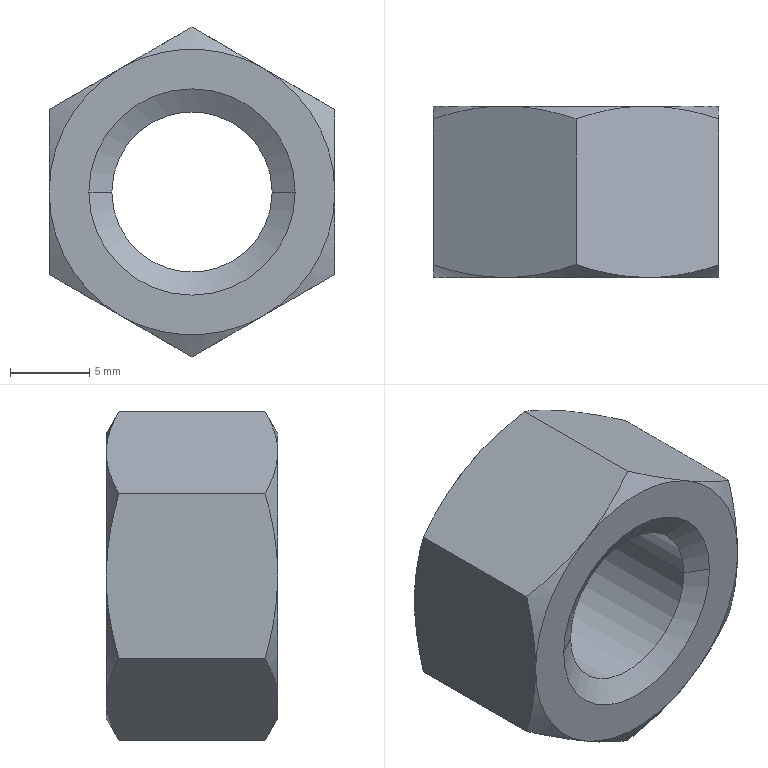Component | SolidWorks | GB_T6170-2015[Type1HexNutM12]-1 | 1 solid | 26 faces | box 18 x 10.8 x 20.78 mm | volume 2109 mm3 | cone 16 | plane 8 | cylinder 2 | commonest cylinder face diameters 10.106 x2
build123d program:
from build123d import *

# Parameters (mm, degrees)
SKETCH3_R           = 5.053
BOSS_EXTRUDE1_DEPTH = 10.8
SKETCH5_R           = 15.023
SKETCH5_R_2         = 9
CUT_EXTRUDE1_DEPTH  = 2.16
CUT_EXTRUDE1_DRAFT  = -60
SKETCH7_R           = 15.023
SKETCH7_R_2         = 9
CUT_EXTRUDE2_DEPTH  = 2.16
CUT_EXTRUDE2_DRAFT  = -60


with BuildPart() as part:
    # Sketch3 → Boss-Extrude1 (new body)
    with BuildSketch(Plane.XY):
        Polygon((0, 10.392), (-9, 5.196), (-9, -5.196), (0, -10.392), (9, -5.196), (9, 5.196), align=None)
        Circle(SKETCH3_R, mode=Mode.SUBTRACT)
    extrude(amount=-BOSS_EXTRUDE1_DEPTH)

    # Sketch4 → Cut-Revolve1 (revolve, cut)
    with BuildSketch(Plane(origin=(0, 0, 0), x_dir=(0, 0, -1), z_dir=(1, 0, 0)), mode=Mode.PRIVATE) as cut_revolve1_sk:
        Polygon((0, 6.5), (0.8355, 5.053), (0.8355, 0), (0, 0), align=None)
        Polygon((10.8, 0), (10.8, 6.5), (9.964, 5.053), (9.964, 0), align=None)
    revolve(cut_revolve1_sk.sketch.rotate(Axis((0, 0, 0), (0, 0, -1)), 90), axis=Axis((0, 0, 0), (0, 0, -1)), mode=Mode.SUBTRACT)


with BuildPart() as cut_extrude1_tool:
    # Sketch5 → Cut-Extrude1 (with draft: the straight prism first)
    with BuildSketch(Plane.XY):
        Circle(SKETCH5_R)
        Circle(SKETCH5_R_2, mode=Mode.SUBTRACT)
    extrude(amount=-CUT_EXTRUDE1_DEPTH)
    # Cut-Extrude1: the draft: its side faces are tilted about the plane it starts from
    cut_extrude1_sides = [cut_extrude1_tool.faces().sort_by_distance(p)[0] for p in [
        (-15.023, 0, -1.08),
        (-9, 0, -1.08),
    ]]
    draft(cut_extrude1_sides, Plane.XY, CUT_EXTRUDE1_DRAFT)


with BuildPart() as part_1:
    add(part.part)

    # Cut-Extrude1: cut by cut_extrude1_tool
    add(cut_extrude1_tool.part, mode=Mode.SUBTRACT)


with BuildPart() as cut_extrude2_tool:
    # Sketch7 → Cut-Extrude2 (with draft: the straight prism first)
    with BuildSketch(Plane(origin=(0, 0, -10.8), x_dir=(-1, 0, 0), z_dir=(0, 0, -1))):
        Circle(SKETCH7_R)
        Circle(SKETCH7_R_2, mode=Mode.SUBTRACT)
    extrude(amount=-CUT_EXTRUDE2_DEPTH)
    # Cut-Extrude2: the draft: its side faces are tilted about the plane it starts from
    cut_extrude2_sides = [cut_extrude2_tool.faces().sort_by_distance(p)[0] for p in [
        (15.023, 0, -9.72),
        (9, 0, -9.72),
    ]]
    draft(cut_extrude2_sides, Plane(origin=(0, 0, -10.8), x_dir=(-1, 0, 0), z_dir=(0, 0, -1)), CUT_EXTRUDE2_DRAFT)


with BuildPart() as part_2:
    add(part_1.part)

    # Cut-Extrude2: cut by cut_extrude2_tool
    add(cut_extrude2_tool.part, mode=Mode.SUBTRACT)


solid = part_2.part

# Placed as in the assembly
solid = solid.moved(Location((128, 179.606, 0), (90, 0, 0)))
STEP:
#1=COLOUR_RGB('',0.7922,0.8196,0.9333);
#2=FILL_AREA_STYLE_COLOUR('',#1);
#3=FILL_AREA_STYLE('',(#2));
#4=SURFACE_STYLE_FILL_AREA(#3);
#5=SURFACE_SIDE_STYLE('',(#4));
#6=SURFACE_STYLE_USAGE(.BOTH.,#5);
#7=PRESENTATION_STYLE_ASSIGNMENT((#6));
#8=CARTESIAN_POINT('',(4.84,7.463,0.));
#9=VERTEX_POINT('',#8);
#10=CARTESIAN_POINT('',(5.238,7.463,0.));
#11=VERTEX_POINT('',#10);
#12=CARTESIAN_POINT('',(5.039,7.463,0.));
#13=DIRECTION('',(0.,-1.,0.));
#14=DIRECTION('',(1.,0.,0.));
#15=AXIS2_PLACEMENT_3D('',#12,#13,#14);
#16=CIRCLE('',#15,0.1989);
#17=EDGE_CURVE('',#9,#11,#16,.T.);
#18=ORIENTED_EDGE('',*,*,#17,.T.);
#19=CARTESIAN_POINT('',(5.295,7.496,0.));
#20=VERTEX_POINT('',#19);
#21=CARTESIAN_POINT('',(5.295,7.496,0.));
#22=DIRECTION('',(0.866,0.5,0.));
#23=VECTOR('',#22,39.37);
#24=LINE('',#21,#23);
#25=EDGE_CURVE('',#11,#20,#24,.T.);
#26=ORIENTED_EDGE('',*,*,#25,.T.);
#27=CARTESIAN_POINT('',(4.783,7.496,0.));
#28=VERTEX_POINT('',#27);
#29=CARTESIAN_POINT('',(5.039,7.496,0.));
#30=DIRECTION('',(0.,-1.,0.));
#31=DIRECTION('',(1.,0.,0.));
#32=AXIS2_PLACEMENT_3D('',#29,#30,#31);
#33=CIRCLE('',#32,0.2559);
#34=EDGE_CURVE('',#28,#20,#33,.T.);
#35=ORIENTED_EDGE('',*,*,#34,.F.);
#36=CARTESIAN_POINT('',(4.783,7.496,0.));
#37=DIRECTION('',(-0.866,0.5,0.));
#38=VECTOR('',#37,39.37);
#39=LINE('',#36,#38);
#40=EDGE_CURVE('',#9,#28,#39,.T.);
#41=ORIENTED_EDGE('',*,*,#40,.F.);
#42=EDGE_LOOP('',(#18,#26,#35,#41));
#43=FACE_OUTER_BOUND('',#42,.T.);
#44=CARTESIAN_POINT('',(5.039,7.496,0.));
#45=DIRECTION('',(0.,1.,0.));
#46=DIRECTION('',(-1.,0.,0.));
#47=AXIS2_PLACEMENT_3D('',#44,#45,#46);
#48=CONICAL_SURFACE('',#47,0.2559,1.047);
#49=ADVANCED_FACE('',(#43),#48,.F.);
#50=CARTESIAN_POINT('',(4.84,7.104,0.));
#51=VERTEX_POINT('',#50);
#52=CARTESIAN_POINT('',(5.238,7.104,0.));
#53=VERTEX_POINT('',#52);
#54=CARTESIAN_POINT('',(5.039,7.104,0.));
#55=DIRECTION('',(0.,-1.,0.));
#56=DIRECTION('',(1.,0.,0.));
#57=AXIS2_PLACEMENT_3D('',#54,#55,#56);
#58=CIRCLE('',#57,0.1989);
#59=EDGE_CURVE('',#51,#53,#58,.T.);
#60=ORIENTED_EDGE('',*,*,#59,.F.);
#61=CARTESIAN_POINT('',(4.783,7.071,0.));
#62=VERTEX_POINT('',#61);
#63=CARTESIAN_POINT('',(4.84,7.104,0.));
#64=DIRECTION('',(-0.866,-0.5,0.));
#65=VECTOR('',#64,39.37);
#66=LINE('',#63,#65);
#67=EDGE_CURVE('',#51,#62,#66,.T.);
#68=ORIENTED_EDGE('',*,*,#67,.T.);
#69=CARTESIAN_POINT('',(5.295,7.071,0.));
#70=VERTEX_POINT('',#69);
#71=CARTESIAN_POINT('',(5.039,7.071,0.));
#72=DIRECTION('',(0.,-1.,0.));
#73=DIRECTION('',(1.,0.,0.));
#74=AXIS2_PLACEMENT_3D('',#71,#72,#73);
#75=CIRCLE('',#74,0.2559);
#76=EDGE_CURVE('',#62,#70,#75,.T.);
#77=ORIENTED_EDGE('',*,*,#76,.T.);
#78=CARTESIAN_POINT('',(5.238,7.104,0.));
#79=DIRECTION('',(0.866,-0.5,0.));
#80=VECTOR('',#79,39.37);
#81=LINE('',#78,#80);
#82=EDGE_CURVE('',#53,#70,#81,.T.);
#83=ORIENTED_EDGE('',*,*,#82,.F.);
#84=EDGE_LOOP('',(#60,#68,#77,#83));
#85=FACE_OUTER_BOUND('',#84,.T.);
#86=CARTESIAN_POINT('',(5.039,7.104,0.));
#87=DIRECTION('',(0.,-1.,0.));
#88=DIRECTION('',(1.,0.,0.));
#89=AXIS2_PLACEMENT_3D('',#86,#87,#88);
#90=CONICAL_SURFACE('',#89,0.1989,1.047);
#91=ADVANCED_FACE('',(#85),#90,.F.);
#92=ORIENTED_EDGE('',*,*,#17,.F.);
#93=CARTESIAN_POINT('',(4.84,7.496,0.));
#94=DIRECTION('',(0.,-1.,0.));
#95=VECTOR('',#94,39.37);
#96=LINE('',#93,#95);
#97=EDGE_CURVE('',#9,#51,#96,.T.);
#98=ORIENTED_EDGE('',*,*,#97,.T.);
#99=ORIENTED_EDGE('',*,*,#59,.T.);
#100=CARTESIAN_POINT('',(5.238,7.496,0.));
#101=DIRECTION('',(0.,-1.,0.));
#102=VECTOR('',#101,39.37);
#103=LINE('',#100,#102);
#104=EDGE_CURVE('',#11,#53,#103,.T.);
#105=ORIENTED_EDGE('',*,*,#104,.F.);
#106=EDGE_LOOP('',(#92,#98,#99,#105));
#107=FACE_OUTER_BOUND('',#106,.T.);
#108=CARTESIAN_POINT('',(5.039,7.496,0.));
#109=DIRECTION('',(0.,-1.,0.));
#110=DIRECTION('',(1.,0.,0.));
#111=AXIS2_PLACEMENT_3D('',#108,#109,#110);
#112=CYLINDRICAL_SURFACE('',#111,0.1989);
#113=ADVANCED_FACE('',(#107),#112,.F.);
#114=CARTESIAN_POINT('',(5.394,7.465,0.2046));
#115=VERTEX_POINT('',#114);
#116=CARTESIAN_POINT('',(5.394,7.103,0.2046));
#117=VERTEX_POINT('',#116);
#118=CARTESIAN_POINT('',(5.394,7.496,0.2046));
#119=DIRECTION('',(0.,-1.,0.));
#120=VECTOR('',#119,39.37);
#121=LINE('',#118,#120);
#122=EDGE_CURVE('',#115,#117,#121,.T.);
#123=ORIENTED_EDGE('',*,*,#122,.F.);
#124=CARTESIAN_POINT('',(5.217,7.496,0.3069));
#125=VERTEX_POINT('',#124);
#126=CARTESIAN_POINT('',(5.394,7.465,0.2046));
#127=CARTESIAN_POINT('',(5.365,7.474,0.2213));
#128=CARTESIAN_POINT('',(5.336,7.482,0.2382));
#129=CARTESIAN_POINT('',(5.277,7.493,0.2722));
#130=CARTESIAN_POINT('',(5.247,7.496,0.2894));
#131=CARTESIAN_POINT('',(5.217,7.496,0.3069));
#132=B_SPLINE_CURVE_WITH_KNOTS('',3,(#126,#127,#128,#129,#130,#131),.UNSPECIFIED.,.F.,.F.,(4,2,4),(0.00000024,0.002629,0.005258),.UNSPECIFIED.);
#133=EDGE_CURVE('',#115,#125,#132,.T.);
#134=ORIENTED_EDGE('',*,*,#133,.T.);
#135=CARTESIAN_POINT('',(5.039,7.465,0.4091));
#136=VERTEX_POINT('',#135);
#137=CARTESIAN_POINT('',(5.217,7.496,0.3069));
#138=CARTESIAN_POINT('',(5.201,7.496,0.3155));
#139=CARTESIAN_POINT('',(5.186,7.496,0.3243));
#140=CARTESIAN_POINT('',(5.157,7.493,0.3415));
#141=CARTESIAN_POINT('',(5.142,7.49,0.3501));
#142=CARTESIAN_POINT('',(5.097,7.482,0.3756));
#143=CARTESIAN_POINT('',(5.068,7.474,0.3925));
#144=CARTESIAN_POINT('',(5.039,7.465,0.4091));
#145=B_SPLINE_CURVE_WITH_KNOTS('',3,(#137,#138,#139,#140,#141,#142,#143,#144),.UNSPECIFIED.,.F.,.F.,(4,2,2,4),(0.005258,0.006567,0.007877,0.0105),.UNSPECIFIED.);
#146=EDGE_CURVE('',#125,#136,#145,.T.);
#147=ORIENTED_EDGE('',*,*,#146,.T.);
#148=CARTESIAN_POINT('',(5.039,7.103,0.4091));
#149=VERTEX_POINT('',#148);
#150=CARTESIAN_POINT('',(5.039,7.496,0.4091));
#151=DIRECTION('',(0.,-1.,0.));
#152=VECTOR('',#151,39.37);
#153=LINE('',#150,#152);
#154=EDGE_CURVE('',#136,#149,#153,.T.);
#155=ORIENTED_EDGE('',*,*,#154,.T.);
#156=CARTESIAN_POINT('',(5.217,7.071,0.3069));
#157=VERTEX_POINT('',#156);
#158=CARTESIAN_POINT('',(5.039,7.103,0.4091));
#159=CARTESIAN_POINT('',(5.068,7.093,0.3924));
#160=CARTESIAN_POINT('',(5.098,7.085,0.3756));
#161=CARTESIAN_POINT('',(5.157,7.074,0.3415));
#162=CARTESIAN_POINT('',(5.186,7.071,0.3243));
#163=CARTESIAN_POINT('',(5.217,7.071,0.3069));
#164=B_SPLINE_CURVE_WITH_KNOTS('',3,(#158,#159,#160,#161,#162,#163),.UNSPECIFIED.,.F.,.F.,(4,2,4),(0.00000024,0.002629,0.005258),.UNSPECIFIED.);
#165=EDGE_CURVE('',#149,#157,#164,.T.);
#166=ORIENTED_EDGE('',*,*,#165,.T.);
#167=CARTESIAN_POINT('',(5.217,7.071,0.3069));
#168=CARTESIAN_POINT('',(5.232,7.071,0.2982));
#169=CARTESIAN_POINT('',(5.247,7.072,0.2895));
#170=CARTESIAN_POINT('',(5.277,7.075,0.2722));
#171=CARTESIAN_POINT('',(5.291,7.077,0.2636));
#172=CARTESIAN_POINT('',(5.336,7.085,0.2381));
#173=CARTESIAN_POINT('',(5.365,7.093,0.2213));
#174=CARTESIAN_POINT('',(5.394,7.103,0.2046));
#175=B_SPLINE_CURVE_WITH_KNOTS('',3,(#167,#168,#169,#170,#171,#172,#173,#174),.UNSPECIFIED.,.F.,.F.,(4,2,2,4),(0.005258,0.006567,0.007877,0.0105),.UNSPECIFIED.);
#176=EDGE_CURVE('',#157,#117,#175,.T.);
#177=ORIENTED_EDGE('',*,*,#176,.T.);
#178=EDGE_LOOP('',(#123,#134,#147,#155,#166,#177));
#179=FACE_OUTER_BOUND('',#178,.T.);
#180=CARTESIAN_POINT('',(5.394,7.496,0.2046));
#181=DIRECTION('',(0.5,0.,0.866));
#182=DIRECTION('',(-0.866,0.,0.5));
#183=AXIS2_PLACEMENT_3D('',#180,#181,#182);
#184=PLANE('',#183);
#185=ADVANCED_FACE('',(#179),#184,.T.);
#186=CARTESIAN_POINT('',(5.394,7.465,-0.2046));
#187=VERTEX_POINT('',#186);
#188=CARTESIAN_POINT('',(5.394,7.103,-0.2046));
#189=VERTEX_POINT('',#188);
#190=CARTESIAN_POINT('',(5.394,7.496,-0.2046));
#191=DIRECTION('',(0.,-1.,0.));
#192=VECTOR('',#191,39.37);
#193=LINE('',#190,#192);
#194=EDGE_CURVE('',#187,#189,#193,.T.);
#195=ORIENTED_EDGE('',*,*,#194,.F.);
#196=CARTESIAN_POINT('',(5.394,7.496,0.));
#197=VERTEX_POINT('',#196);
#198=CARTESIAN_POINT('',(5.394,7.465,-0.2046));
#199=CARTESIAN_POINT('',(5.394,7.474,-0.1713));
#200=CARTESIAN_POINT('',(5.394,7.482,-0.1372));
#201=CARTESIAN_POINT('',(5.394,7.493,-0.06893));
#202=CARTESIAN_POINT('',(5.394,7.496,-0.03459));
#203=CARTESIAN_POINT('',(5.394,7.496,0.));
#204=B_SPLINE_CURVE_WITH_KNOTS('',3,(#198,#199,#200,#201,#202,#203),.UNSPECIFIED.,.F.,.F.,(4,2,4),(0.009415,0.01204,0.01467),.UNSPECIFIED.);
#205=EDGE_CURVE('',#187,#197,#204,.T.);
#206=ORIENTED_EDGE('',*,*,#205,.T.);
#207=CARTESIAN_POINT('',(5.394,7.496,0.));
#208=CARTESIAN_POINT('',(5.394,7.496,0.03461));
#209=CARTESIAN_POINT('',(5.394,7.493,0.06968));
#210=CARTESIAN_POINT('',(5.394,7.482,0.138));
#211=CARTESIAN_POINT('',(5.394,7.474,0.1715));
#212=CARTESIAN_POINT('',(5.394,7.465,0.2046));
#213=B_SPLINE_CURVE_WITH_KNOTS('',3,(#207,#208,#209,#210,#211,#212),.UNSPECIFIED.,.F.,.F.,(4,2,4),(0.01467,0.0173,0.01993),.UNSPECIFIED.);
#214=EDGE_CURVE('',#197,#115,#213,.T.);
#215=ORIENTED_EDGE('',*,*,#214,.T.);
#216=ORIENTED_EDGE('',*,*,#122,.T.);
#217=CARTESIAN_POINT('',(5.394,7.071,0.));
#218=VERTEX_POINT('',#217);
#219=CARTESIAN_POINT('',(5.394,7.103,0.2046));
#220=CARTESIAN_POINT('',(5.394,7.093,0.1715));
#221=CARTESIAN_POINT('',(5.394,7.085,0.138));
#222=CARTESIAN_POINT('',(5.394,7.074,0.06968));
#223=CARTESIAN_POINT('',(5.394,7.071,0.03461));
#224=CARTESIAN_POINT('',(5.394,7.071,0.));
#225=B_SPLINE_CURVE_WITH_KNOTS('',3,(#219,#220,#221,#222,#223,#224),.UNSPECIFIED.,.F.,.F.,(4,2,4),(0.02316,0.02579,0.02842),.UNSPECIFIED.);
#226=EDGE_CURVE('',#117,#218,#225,.T.);
#227=ORIENTED_EDGE('',*,*,#226,.T.);
#228=CARTESIAN_POINT('',(5.394,7.071,0.));
#229=CARTESIAN_POINT('',(5.394,7.071,-0.03459));
#230=CARTESIAN_POINT('',(5.394,7.074,-0.06893));
#231=CARTESIAN_POINT('',(5.394,7.085,-0.1372));
#232=CARTESIAN_POINT('',(5.394,7.093,-0.1713));
#233=CARTESIAN_POINT('',(5.394,7.103,-0.2046));
#234=B_SPLINE_CURVE_WITH_KNOTS('',3,(#228,#229,#230,#231,#232,#233),.UNSPECIFIED.,.F.,.F.,(4,2,4),(0.02842,0.03105,0.03369),.UNSPECIFIED.);
#235=EDGE_CURVE('',#218,#189,#234,.T.);
#236=ORIENTED_EDGE('',*,*,#235,.T.);
#237=EDGE_LOOP('',(#195,#206,#215,#216,#227,#236));
#238=FACE_OUTER_BOUND('',#237,.T.);
#239=CARTESIAN_POINT('',(5.394,7.496,-0.2046));
#240=DIRECTION('',(1.,0.,0.));
#241=DIRECTION('',(-0.,0.,1.));
#242=AXIS2_PLACEMENT_3D('',#239,#240,#241);
#243=PLANE('',#242);
#244=ADVANCED_FACE('',(#238),#243,.T.);
#245=CARTESIAN_POINT('',(5.039,7.465,-0.4091));
#246=VERTEX_POINT('',#245);
#247=CARTESIAN_POINT('',(5.039,7.103,-0.4091));
#248=VERTEX_POINT('',#247);
#249=CARTESIAN_POINT('',(5.039,7.496,-0.4091));
#250=DIRECTION('',(0.,-1.,0.));
#251=VECTOR('',#250,39.37);
#252=LINE('',#249,#251);
#253=EDGE_CURVE('',#246,#248,#252,.T.);
#254=ORIENTED_EDGE('',*,*,#253,.F.);
#255=CARTESIAN_POINT('',(5.217,7.496,-0.3069));
#256=VERTEX_POINT('',#255);
#257=CARTESIAN_POINT('',(5.039,7.465,-0.4091));
#258=CARTESIAN_POINT('',(5.068,7.474,-0.3924));
#259=CARTESIAN_POINT('',(5.098,7.482,-0.3756));
#260=CARTESIAN_POINT('',(5.157,7.493,-0.3415));
#261=CARTESIAN_POINT('',(5.186,7.496,-0.3243));
#262=CARTESIAN_POINT('',(5.217,7.496,-0.3069));
#263=B_SPLINE_CURVE_WITH_KNOTS('',3,(#257,#258,#259,#260,#261,#262),.UNSPECIFIED.,.F.,.F.,(4,2,4),(0.00000024,0.002629,0.005258),.UNSPECIFIED.);
#264=EDGE_CURVE('',#246,#256,#263,.T.);
#265=ORIENTED_EDGE('',*,*,#264,.T.);
#266=CARTESIAN_POINT('',(5.217,7.496,-0.3069));
#267=CARTESIAN_POINT('',(5.232,7.496,-0.2982));
#268=CARTESIAN_POINT('',(5.247,7.496,-0.2895));
#269=CARTESIAN_POINT('',(5.277,7.493,-0.2722));
#270=CARTESIAN_POINT('',(5.291,7.49,-0.2636));
#271=CARTESIAN_POINT('',(5.336,7.482,-0.2381));
#272=CARTESIAN_POINT('',(5.365,7.474,-0.2213));
#273=CARTESIAN_POINT('',(5.394,7.465,-0.2046));
#274=B_SPLINE_CURVE_WITH_KNOTS('',3,(#266,#267,#268,#269,#270,#271,#272,#273),.UNSPECIFIED.,.F.,.F.,(4,2,2,4),(0.005258,0.006567,0.007877,0.0105),.UNSPECIFIED.);
#275=EDGE_CURVE('',#256,#187,#274,.T.);
#276=ORIENTED_EDGE('',*,*,#275,.T.);
#277=ORIENTED_EDGE('',*,*,#194,.T.);
#278=CARTESIAN_POINT('',(5.217,7.071,-0.3069));
#279=VERTEX_POINT('',#278);
#280=CARTESIAN_POINT('',(5.394,7.103,-0.2046));
#281=CARTESIAN_POINT('',(5.365,7.093,-0.2213));
#282=CARTESIAN_POINT('',(5.336,7.085,-0.2382));
#283=CARTESIAN_POINT('',(5.277,7.074,-0.2722));
#284=CARTESIAN_POINT('',(5.247,7.071,-0.2894));
#285=CARTESIAN_POINT('',(5.217,7.071,-0.3069));
#286=B_SPLINE_CURVE_WITH_KNOTS('',3,(#280,#281,#282,#283,#284,#285),.UNSPECIFIED.,.F.,.F.,(4,2,4),(0.00000024,0.002629,0.005258),.UNSPECIFIED.);
#287=EDGE_CURVE('',#189,#279,#286,.T.);
#288=ORIENTED_EDGE('',*,*,#287,.T.);
#289=CARTESIAN_POINT('',(5.217,7.071,-0.3069));
#290=CARTESIAN_POINT('',(5.201,7.071,-0.3155));
#291=CARTESIAN_POINT('',(5.186,7.072,-0.3243));
#292=CARTESIAN_POINT('',(5.157,7.075,-0.3415));
#293=CARTESIAN_POINT('',(5.142,7.077,-0.3501));
#294=CARTESIAN_POINT('',(5.097,7.085,-0.3756));
#295=CARTESIAN_POINT('',(5.068,7.093,-0.3925));
#296=CARTESIAN_POINT('',(5.039,7.103,-0.4091));
#297=B_SPLINE_CURVE_WITH_KNOTS('',3,(#289,#290,#291,#292,#293,#294,#295,#296),.UNSPECIFIED.,.F.,.F.,(4,2,2,4),(0.005258,0.006567,0.007877,0.0105),.UNSPECIFIED.);
#298=EDGE_CURVE('',#279,#248,#297,.T.);
#299=ORIENTED_EDGE('',*,*,#298,.T.);
#300=EDGE_LOOP('',(#254,#265,#276,#277,#288,#299));
#301=FACE_OUTER_BOUND('',#300,.T.);
#302=CARTESIAN_POINT('',(5.039,7.496,-0.4091));
#303=DIRECTION('',(0.5,0.,-0.866));
#304=DIRECTION('',(0.866,0.,0.5));
#305=AXIS2_PLACEMENT_3D('',#302,#303,#304);
#306=PLANE('',#305);
#307=ADVANCED_FACE('',(#301),#306,.T.);
#308=CARTESIAN_POINT('',(4.685,7.465,-0.2046));
#309=VERTEX_POINT('',#308);
#310=CARTESIAN_POINT('',(4.685,7.103,-0.2046));
#311=VERTEX_POINT('',#310);
#312=CARTESIAN_POINT('',(4.685,7.496,-0.2046));
#313=DIRECTION('',(0.,-1.,0.));
#314=VECTOR('',#313,39.37);
#315=LINE('',#312,#314);
#316=EDGE_CURVE('',#309,#311,#315,.T.);
#317=ORIENTED_EDGE('',*,*,#316,.F.);
#318=CARTESIAN_POINT('',(4.862,7.496,-0.3069));
#319=VERTEX_POINT('',#318);
#320=CARTESIAN_POINT('',(4.685,7.465,-0.2046));
#321=CARTESIAN_POINT('',(4.714,7.474,-0.2213));
#322=CARTESIAN_POINT('',(4.743,7.482,-0.2382));
#323=CARTESIAN_POINT('',(4.802,7.493,-0.2722));
#324=CARTESIAN_POINT('',(4.832,7.496,-0.2894));
#325=CARTESIAN_POINT('',(4.862,7.496,-0.3069));
#326=B_SPLINE_CURVE_WITH_KNOTS('',3,(#320,#321,#322,#323,#324,#325),.UNSPECIFIED.,.F.,.F.,(4,2,4),(0.00000024,0.002629,0.005258),.UNSPECIFIED.);
#327=EDGE_CURVE('',#309,#319,#326,.T.);
#328=ORIENTED_EDGE('',*,*,#327,.T.);
#329=CARTESIAN_POINT('',(4.862,7.496,-0.3069));
#330=CARTESIAN_POINT('',(4.877,7.496,-0.3155));
#331=CARTESIAN_POINT('',(4.892,7.496,-0.3243));
#332=CARTESIAN_POINT('',(4.922,7.493,-0.3415));
#333=CARTESIAN_POINT('',(4.937,7.49,-0.3501));
#334=CARTESIAN_POINT('',(4.981,7.482,-0.3756));
#335=CARTESIAN_POINT('',(5.01,7.474,-0.3925));
#336=CARTESIAN_POINT('',(5.039,7.465,-0.4091));
#337=B_SPLINE_CURVE_WITH_KNOTS('',3,(#329,#330,#331,#332,#333,#334,#335,#336),.UNSPECIFIED.,.F.,.F.,(4,2,2,4),(0.005258,0.006567,0.007877,0.0105),.UNSPECIFIED.);
#338=EDGE_CURVE('',#319,#246,#337,.T.);
#339=ORIENTED_EDGE('',*,*,#338,.T.);
#340=ORIENTED_EDGE('',*,*,#253,.T.);
#341=CARTESIAN_POINT('',(4.862,7.071,-0.3069));
#342=VERTEX_POINT('',#341);
#343=CARTESIAN_POINT('',(5.039,7.103,-0.4091));
#344=CARTESIAN_POINT('',(5.01,7.093,-0.3924));
#345=CARTESIAN_POINT('',(4.981,7.085,-0.3756));
#346=CARTESIAN_POINT('',(4.922,7.074,-0.3415));
#347=CARTESIAN_POINT('',(4.892,7.071,-0.3243));
#348=CARTESIAN_POINT('',(4.862,7.071,-0.3069));
#349=B_SPLINE_CURVE_WITH_KNOTS('',3,(#343,#344,#345,#346,#347,#348),.UNSPECIFIED.,.F.,.F.,(4,2,4),(0.00000024,0.002629,0.005258),.UNSPECIFIED.);
#350=EDGE_CURVE('',#248,#342,#349,.T.);
#351=ORIENTED_EDGE('',*,*,#350,.T.);
#352=CARTESIAN_POINT('',(4.862,7.071,-0.3069));
#353=CARTESIAN_POINT('',(4.847,7.071,-0.2982));
#354=CARTESIAN_POINT('',(4.832,7.072,-0.2895));
#355=CARTESIAN_POINT('',(4.802,7.075,-0.2722));
#356=CARTESIAN_POINT('',(4.787,7.077,-0.2636));
#357=CARTESIAN_POINT('',(4.743,7.085,-0.2381));
#358=CARTESIAN_POINT('',(4.714,7.093,-0.2213));
#359=CARTESIAN_POINT('',(4.685,7.103,-0.2046));
#360=B_SPLINE_CURVE_WITH_KNOTS('',3,(#352,#353,#354,#355,#356,#357,#358,#359),.UNSPECIFIED.,.F.,.F.,(4,2,2,4),(0.005258,0.006567,0.007877,0.0105),.UNSPECIFIED.);
#361=EDGE_CURVE('',#342,#311,#360,.T.);
#362=ORIENTED_EDGE('',*,*,#361,.T.);
#363=EDGE_LOOP('',(#317,#328,#339,#340,#351,#362));
#364=FACE_OUTER_BOUND('',#363,.T.);
#365=CARTESIAN_POINT('',(4.685,7.496,-0.2046));
#366=DIRECTION('',(-0.5,0.,-0.866));
#367=DIRECTION('',(0.866,0.,-0.5));
#368=AXIS2_PLACEMENT_3D('',#365,#366,#367);
#369=PLANE('',#368);
#370=ADVANCED_FACE('',(#364),#369,.T.);
#371=CARTESIAN_POINT('',(4.685,7.465,0.2046));
#372=VERTEX_POINT('',#371);
#373=CARTESIAN_POINT('',(4.685,7.103,0.2046));
#374=VERTEX_POINT('',#373);
#375=CARTESIAN_POINT('',(4.685,7.496,0.2046));
#376=DIRECTION('',(0.,-1.,0.));
#377=VECTOR('',#376,39.37);
#378=LINE('',#375,#377);
#379=EDGE_CURVE('',#372,#374,#378,.T.);
#380=ORIENTED_EDGE('',*,*,#379,.F.);
#381=CARTESIAN_POINT('',(4.685,7.496,0.));
#382=VERTEX_POINT('',#381);
#383=CARTESIAN_POINT('',(4.685,7.465,0.2046));
#384=CARTESIAN_POINT('',(4.685,7.474,0.1715));
#385=CARTESIAN_POINT('',(4.685,7.482,0.138));
#386=CARTESIAN_POINT('',(4.685,7.493,0.06968));
#387=CARTESIAN_POINT('',(4.685,7.496,0.03461));
#388=CARTESIAN_POINT('',(4.685,7.496,0.));
#389=B_SPLINE_CURVE_WITH_KNOTS('',3,(#383,#384,#385,#386,#387,#388),.UNSPECIFIED.,.F.,.F.,(4,2,4),(0.02316,0.02579,0.02842),.UNSPECIFIED.);
#390=EDGE_CURVE('',#372,#382,#389,.T.);
#391=ORIENTED_EDGE('',*,*,#390,.T.);
#392=CARTESIAN_POINT('',(4.685,7.496,0.));
#393=CARTESIAN_POINT('',(4.685,7.496,-0.03459));
#394=CARTESIAN_POINT('',(4.685,7.493,-0.06893));
#395=CARTESIAN_POINT('',(4.685,7.482,-0.1372));
#396=CARTESIAN_POINT('',(4.685,7.474,-0.1713));
#397=CARTESIAN_POINT('',(4.685,7.465,-0.2046));
#398=B_SPLINE_CURVE_WITH_KNOTS('',3,(#392,#393,#394,#395,#396,#397),.UNSPECIFIED.,.F.,.F.,(4,2,4),(0.02842,0.03105,0.03369),.UNSPECIFIED.);
#399=EDGE_CURVE('',#382,#309,#398,.T.);
#400=ORIENTED_EDGE('',*,*,#399,.T.);
#401=ORIENTED_EDGE('',*,*,#316,.T.);
#402=CARTESIAN_POINT('',(4.685,7.071,0.));
#403=VERTEX_POINT('',#402);
#404=CARTESIAN_POINT('',(4.685,7.103,-0.2046));
#405=CARTESIAN_POINT('',(4.685,7.093,-0.1713));
#406=CARTESIAN_POINT('',(4.685,7.085,-0.1372));
#407=CARTESIAN_POINT('',(4.685,7.074,-0.06893));
#408=CARTESIAN_POINT('',(4.685,7.071,-0.03459));
#409=CARTESIAN_POINT('',(4.685,7.071,0.));
#410=B_SPLINE_CURVE_WITH_KNOTS('',3,(#404,#405,#406,#407,#408,#409),.UNSPECIFIED.,.F.,.F.,(4,2,4),(0.009415,0.01204,0.01467),.UNSPECIFIED.);
#411=EDGE_CURVE('',#311,#403,#410,.T.);
#412=ORIENTED_EDGE('',*,*,#411,.T.);
#413=CARTESIAN_POINT('',(4.685,7.071,0.));
#414=CARTESIAN_POINT('',(4.685,7.071,0.03461));
#415=CARTESIAN_POINT('',(4.685,7.074,0.06968));
#416=CARTESIAN_POINT('',(4.685,7.085,0.138));
#417=CARTESIAN_POINT('',(4.685,7.093,0.1715));
#418=CARTESIAN_POINT('',(4.685,7.103,0.2046));
#419=B_SPLINE_CURVE_WITH_KNOTS('',3,(#413,#414,#415,#416,#417,#418),.UNSPECIFIED.,.F.,.F.,(4,2,4),(0.01467,0.0173,0.01993),.UNSPECIFIED.);
#420=EDGE_CURVE('',#403,#374,#419,.T.);
#421=ORIENTED_EDGE('',*,*,#420,.T.);
#422=EDGE_LOOP('',(#380,#391,#400,#401,#412,#421));
#423=FACE_OUTER_BOUND('',#422,.T.);
#424=CARTESIAN_POINT('',(4.685,7.496,0.2046));
#425=DIRECTION('',(-1.,0.,0.));
#426=DIRECTION('',(0.,-1.,0.));
#427=AXIS2_PLACEMENT_3D('',#424,#425,#426);
#428=PLANE('',#427);
#429=ADVANCED_FACE('',(#423),#428,.T.);
#430=ORIENTED_EDGE('',*,*,#154,.F.);
#431=CARTESIAN_POINT('',(4.862,7.496,0.3069));
#432=VERTEX_POINT('',#431);
#433=CARTESIAN_POINT('',(5.039,7.465,0.4091));
#434=CARTESIAN_POINT('',(5.01,7.474,0.3924));
#435=CARTESIAN_POINT('',(4.981,7.482,0.3756));
#436=CARTESIAN_POINT('',(4.922,7.493,0.3415));
#437=CARTESIAN_POINT('',(4.892,7.496,0.3243));
#438=CARTESIAN_POINT('',(4.862,7.496,0.3069));
#439=B_SPLINE_CURVE_WITH_KNOTS('',3,(#433,#434,#435,#436,#437,#438),.UNSPECIFIED.,.F.,.F.,(4,2,4),(0.00000024,0.002629,0.005258),.UNSPECIFIED.);
#440=EDGE_CURVE('',#136,#432,#439,.T.);
#441=ORIENTED_EDGE('',*,*,#440,.T.);
#442=CARTESIAN_POINT('',(4.862,7.496,0.3069));
#443=CARTESIAN_POINT('',(4.847,7.496,0.2982));
#444=CARTESIAN_POINT('',(4.832,7.496,0.2895));
#445=CARTESIAN_POINT('',(4.802,7.493,0.2722));
#446=CARTESIAN_POINT('',(4.787,7.49,0.2636));
#447=CARTESIAN_POINT('',(4.743,7.482,0.2381));
#448=CARTESIAN_POINT('',(4.714,7.474,0.2213));
#449=CARTESIAN_POINT('',(4.685,7.465,0.2046));
#450=B_SPLINE_CURVE_WITH_KNOTS('',3,(#442,#443,#444,#445,#446,#447,#448,#449),.UNSPECIFIED.,.F.,.F.,(4,2,2,4),(0.005258,0.006567,0.007877,0.0105),.UNSPECIFIED.);
#451=EDGE_CURVE('',#432,#372,#450,.T.);
#452=ORIENTED_EDGE('',*,*,#451,.T.);
#453=ORIENTED_EDGE('',*,*,#379,.T.);
#454=CARTESIAN_POINT('',(4.862,7.071,0.3069));
#455=VERTEX_POINT('',#454);
#456=CARTESIAN_POINT('',(4.685,7.103,0.2046));
#457=CARTESIAN_POINT('',(4.714,7.093,0.2213));
#458=CARTESIAN_POINT('',(4.743,7.085,0.2382));
#459=CARTESIAN_POINT('',(4.802,7.074,0.2722));
#460=CARTESIAN_POINT('',(4.832,7.071,0.2894));
#461=CARTESIAN_POINT('',(4.862,7.071,0.3069));
#462=B_SPLINE_CURVE_WITH_KNOTS('',3,(#456,#457,#458,#459,#460,#461),.UNSPECIFIED.,.F.,.F.,(4,2,4),(0.00000024,0.002629,0.005258),.UNSPECIFIED.);
#463=EDGE_CURVE('',#374,#455,#462,.T.);
#464=ORIENTED_EDGE('',*,*,#463,.T.);
#465=CARTESIAN_POINT('',(4.862,7.071,0.3069));
#466=CARTESIAN_POINT('',(4.877,7.071,0.3155));
#467=CARTESIAN_POINT('',(4.892,7.072,0.3243));
#468=CARTESIAN_POINT('',(4.922,7.075,0.3415));
#469=CARTESIAN_POINT('',(4.937,7.077,0.3501));
#470=CARTESIAN_POINT('',(4.981,7.085,0.3756));
#471=CARTESIAN_POINT('',(5.01,7.093,0.3925));
#472=CARTESIAN_POINT('',(5.039,7.103,0.4091));
#473=B_SPLINE_CURVE_WITH_KNOTS('',3,(#465,#466,#467,#468,#469,#470,#471,#472),.UNSPECIFIED.,.F.,.F.,(4,2,2,4),(0.005258,0.006567,0.007877,0.0105),.UNSPECIFIED.);
#474=EDGE_CURVE('',#455,#149,#473,.T.);
#475=ORIENTED_EDGE('',*,*,#474,.T.);
#476=EDGE_LOOP('',(#430,#441,#452,#453,#464,#475));
#477=FACE_OUTER_BOUND('',#476,.T.);
#478=CARTESIAN_POINT('',(5.039,7.496,0.4091));
#479=DIRECTION('',(-0.5,0.,0.866));
#480=DIRECTION('',(-0.866,0.,-0.5));
#481=AXIS2_PLACEMENT_3D('',#478,#479,#480);
#482=PLANE('',#481);
#483=ADVANCED_FACE('',(#477),#482,.T.);
#484=ORIENTED_EDGE('',*,*,#34,.T.);
#485=CARTESIAN_POINT('',(5.039,7.496,0.));
#486=DIRECTION('',(0.,-1.,0.));
#487=DIRECTION('',(1.,0.,0.));
#488=AXIS2_PLACEMENT_3D('',#485,#486,#487);
#489=CIRCLE('',#488,0.2559);
#490=EDGE_CURVE('',#20,#28,#489,.T.);
#491=ORIENTED_EDGE('',*,*,#490,.T.);
#492=EDGE_LOOP('',(#484,#491));
#493=FACE_BOUND('',#492,.T.);
#494=CARTESIAN_POINT('',(5.039,7.496,0.));
#495=DIRECTION('',(0.,-1.,0.));
#496=DIRECTION('',(1.,0.,0.));
#497=AXIS2_PLACEMENT_3D('',#494,#495,#496);
#498=CIRCLE('',#497,0.3543);
#499=EDGE_CURVE('',#197,#125,#498,.T.);
#500=ORIENTED_EDGE('',*,*,#499,.F.);
#501=CARTESIAN_POINT('',(5.039,7.496,0.));
#502=DIRECTION('',(0.,-1.,0.));
#503=DIRECTION('',(1.,0.,0.));
#504=AXIS2_PLACEMENT_3D('',#501,#502,#503);
#505=CIRCLE('',#504,0.3543);
#506=EDGE_CURVE('',#256,#197,#505,.T.);
#507=ORIENTED_EDGE('',*,*,#506,.F.);
#508=CARTESIAN_POINT('',(5.039,7.496,0.));
#509=DIRECTION('',(0.,-1.,0.));
#510=DIRECTION('',(1.,0.,0.));
#511=AXIS2_PLACEMENT_3D('',#508,#509,#510);
#512=CIRCLE('',#511,0.3543);
#513=EDGE_CURVE('',#319,#256,#512,.T.);
#514=ORIENTED_EDGE('',*,*,#513,.F.);
#515=CARTESIAN_POINT('',(5.039,7.496,0.));
#516=DIRECTION('',(0.,-1.,0.));
#517=DIRECTION('',(1.,0.,0.));
#518=AXIS2_PLACEMENT_3D('',#515,#516,#517);
#519=CIRCLE('',#518,0.3543);
#520=EDGE_CURVE('',#382,#319,#519,.T.);
#521=ORIENTED_EDGE('',*,*,#520,.F.);
#522=CARTESIAN_POINT('',(5.039,7.496,0.));
#523=DIRECTION('',(0.,1.,0.));
#524=DIRECTION('',(-1.,0.,0.));
#525=AXIS2_PLACEMENT_3D('',#522,#523,#524);
#526=CIRCLE('',#525,0.3543);
#527=EDGE_CURVE('',#382,#432,#526,.T.);
#528=ORIENTED_EDGE('',*,*,#527,.T.);
#529=CARTESIAN_POINT('',(5.039,7.496,0.));
#530=DIRECTION('',(0.,-1.,0.));
#531=DIRECTION('',(1.,0.,0.));
#532=AXIS2_PLACEMENT_3D('',#529,#530,#531);
#533=CIRCLE('',#532,0.3543);
#534=EDGE_CURVE('',#125,#432,#533,.T.);
#535=ORIENTED_EDGE('',*,*,#534,.F.);
#536=EDGE_LOOP('',(#500,#507,#514,#521,#528,#535));
#537=FACE_OUTER_BOUND('',#536,.T.);
#538=CARTESIAN_POINT('',(5.039,7.496,0.4091));
#539=DIRECTION('',(0.,-1.,0.));
#540=DIRECTION('',(1.,0.,0.));
#541=AXIS2_PLACEMENT_3D('',#538,#539,#540);
#542=PLANE('',#541);
#543=ADVANCED_FACE('',(#493,#537),#542,.F.);
#544=CARTESIAN_POINT('',(5.039,7.071,0.));
#545=DIRECTION('',(0.,-1.,0.));
#546=DIRECTION('',(1.,0.,0.));
#547=AXIS2_PLACEMENT_3D('',#544,#545,#546);
#548=CIRCLE('',#547,0.2559);
#549=EDGE_CURVE('',#70,#62,#548,.T.);
#550=ORIENTED_EDGE('',*,*,#549,.F.);
#551=ORIENTED_EDGE('',*,*,#76,.F.);
#552=EDGE_LOOP('',(#550,#551));
#553=FACE_BOUND('',#552,.T.);
#554=CARTESIAN_POINT('',(5.039,7.071,0.));
#555=DIRECTION('',(0.,-1.,0.));
#556=DIRECTION('',(1.,0.,0.));
#557=AXIS2_PLACEMENT_3D('',#554,#555,#556);
#558=CIRCLE('',#557,0.3543);
#559=EDGE_CURVE('',#279,#218,#558,.T.);
#560=ORIENTED_EDGE('',*,*,#559,.T.);
#561=CARTESIAN_POINT('',(5.039,7.071,0.));
#562=DIRECTION('',(0.,-1.,0.));
#563=DIRECTION('',(1.,0.,0.));
#564=AXIS2_PLACEMENT_3D('',#561,#562,#563);
#565=CIRCLE('',#564,0.3543);
#566=EDGE_CURVE('',#218,#157,#565,.T.);
#567=ORIENTED_EDGE('',*,*,#566,.T.);
#568=CARTESIAN_POINT('',(5.039,7.071,0.));
#569=DIRECTION('',(0.,-1.,0.));
#570=DIRECTION('',(1.,0.,0.));
#571=AXIS2_PLACEMENT_3D('',#568,#569,#570);
#572=CIRCLE('',#571,0.3543);
#573=EDGE_CURVE('',#157,#455,#572,.T.);
#574=ORIENTED_EDGE('',*,*,#573,.T.);
#575=CARTESIAN_POINT('',(5.039,7.071,0.));
#576=DIRECTION('',(0.,-1.,0.));
#577=DIRECTION('',(1.,0.,0.));
#578=AXIS2_PLACEMENT_3D('',#575,#576,#577);
#579=CIRCLE('',#578,0.3543);
#580=EDGE_CURVE('',#455,#403,#579,.T.);
#581=ORIENTED_EDGE('',*,*,#580,.T.);
#582=CARTESIAN_POINT('',(5.039,7.071,0.));
#583=DIRECTION('',(0.,-1.,0.));
#584=DIRECTION('',(1.,0.,0.));
#585=AXIS2_PLACEMENT_3D('',#582,#583,#584);
#586=CIRCLE('',#585,0.3543);
#587=EDGE_CURVE('',#403,#342,#586,.T.);
#588=ORIENTED_EDGE('',*,*,#587,.T.);
#589=CARTESIAN_POINT('',(5.039,7.071,0.));
#590=DIRECTION('',(0.,-1.,0.));
#591=DIRECTION('',(1.,0.,0.));
#592=AXIS2_PLACEMENT_3D('',#589,#590,#591);
#593=CIRCLE('',#592,0.3543);
#594=EDGE_CURVE('',#342,#279,#593,.T.);
#595=ORIENTED_EDGE('',*,*,#594,.T.);
#596=EDGE_LOOP('',(#560,#567,#574,#581,#588,#595));
#597=FACE_OUTER_BOUND('',#596,.T.);
#598=CARTESIAN_POINT('',(5.039,7.071,0.4091));
#599=DIRECTION('',(0.,-1.,0.));
#600=DIRECTION('',(1.,0.,0.));
#601=AXIS2_PLACEMENT_3D('',#598,#599,#600);
#602=PLANE('',#601);
#603=ADVANCED_FACE('',(#553,#597),#602,.T.);
#604=ORIENTED_EDGE('',*,*,#97,.F.);
#605=CARTESIAN_POINT('',(5.039,7.463,0.));
#606=DIRECTION('',(0.,-1.,0.));
#607=DIRECTION('',(1.,0.,0.));
#608=AXIS2_PLACEMENT_3D('',#605,#606,#607);
#609=CIRCLE('',#608,0.1989);
#610=EDGE_CURVE('',#11,#9,#609,.T.);
#611=ORIENTED_EDGE('',*,*,#610,.F.);
#612=ORIENTED_EDGE('',*,*,#104,.T.);
#613=CARTESIAN_POINT('',(5.039,7.104,0.));
#614=DIRECTION('',(0.,-1.,0.));
#615=DIRECTION('',(1.,0.,0.));
#616=AXIS2_PLACEMENT_3D('',#613,#614,#615);
#617=CIRCLE('',#616,0.1989);
#618=EDGE_CURVE('',#53,#51,#617,.T.);
#619=ORIENTED_EDGE('',*,*,#618,.T.);
#620=EDGE_LOOP('',(#604,#611,#612,#619));
#621=FACE_OUTER_BOUND('',#620,.T.);
#622=CARTESIAN_POINT('',(5.039,7.496,0.));
#623=DIRECTION('',(0.,-1.,0.));
#624=DIRECTION('',(1.,0.,0.));
#625=AXIS2_PLACEMENT_3D('',#622,#623,#624);
#626=CYLINDRICAL_SURFACE('',#625,0.1989);
#627=ADVANCED_FACE('',(#621),#626,.F.);
#628=ORIENTED_EDGE('',*,*,#67,.F.);
#629=ORIENTED_EDGE('',*,*,#618,.F.);
#630=ORIENTED_EDGE('',*,*,#82,.T.);
#631=ORIENTED_EDGE('',*,*,#549,.T.);
#632=EDGE_LOOP('',(#628,#629,#630,#631));
#633=FACE_OUTER_BOUND('',#632,.T.);
#634=CARTESIAN_POINT('',(5.039,7.104,0.));
#635=DIRECTION('',(0.,-1.,0.));
#636=DIRECTION('',(1.,0.,0.));
#637=AXIS2_PLACEMENT_3D('',#634,#635,#636);
#638=CONICAL_SURFACE('',#637,0.1989,1.047);
#639=ADVANCED_FACE('',(#633),#638,.F.);
#640=ORIENTED_EDGE('',*,*,#25,.F.);
#641=ORIENTED_EDGE('',*,*,#610,.T.);
#642=ORIENTED_EDGE('',*,*,#40,.T.);
#643=ORIENTED_EDGE('',*,*,#490,.F.);
#644=EDGE_LOOP('',(#640,#641,#642,#643));
#645=FACE_OUTER_BOUND('',#644,.T.);
#646=CARTESIAN_POINT('',(5.039,7.496,0.));
#647=DIRECTION('',(0.,1.,0.));
#648=DIRECTION('',(-1.,0.,0.));
#649=AXIS2_PLACEMENT_3D('',#646,#647,#648);
#650=CONICAL_SURFACE('',#649,0.2559,1.047);
#651=ADVANCED_FACE('',(#645),#650,.F.);
#652=ORIENTED_EDGE('',*,*,#474,.F.);
#653=ORIENTED_EDGE('',*,*,#573,.F.);
#654=ORIENTED_EDGE('',*,*,#165,.F.);
#655=EDGE_LOOP('',(#652,#653,#654));
#656=FACE_OUTER_BOUND('',#655,.T.);
#657=CARTESIAN_POINT('',(5.039,7.071,0.));
#658=DIRECTION('',(0.,1.,0.));
#659=DIRECTION('',(1.,0.,0.));
#660=AXIS2_PLACEMENT_3D('',#657,#658,#659);
#661=CONICAL_SURFACE('',#660,0.3543,1.047);
#662=ADVANCED_FACE('',(#656),#661,.T.);
#663=ORIENTED_EDGE('',*,*,#580,.F.);
#664=ORIENTED_EDGE('',*,*,#463,.F.);
#665=ORIENTED_EDGE('',*,*,#420,.F.);
#666=EDGE_LOOP('',(#663,#664,#665));
#667=FACE_OUTER_BOUND('',#666,.T.);
#668=CARTESIAN_POINT('',(5.039,7.071,0.));
#669=DIRECTION('',(0.,1.,0.));
#670=DIRECTION('',(1.,0.,0.));
#671=AXIS2_PLACEMENT_3D('',#668,#669,#670);
#672=CONICAL_SURFACE('',#671,0.3543,1.047);
#673=ADVANCED_FACE('',(#667),#672,.T.);
#674=ORIENTED_EDGE('',*,*,#587,.F.);
#675=ORIENTED_EDGE('',*,*,#411,.F.);
#676=ORIENTED_EDGE('',*,*,#361,.F.);
#677=EDGE_LOOP('',(#674,#675,#676));
#678=FACE_OUTER_BOUND('',#677,.T.);
#679=CARTESIAN_POINT('',(5.039,7.071,0.));
#680=DIRECTION('',(0.,1.,0.));
#681=DIRECTION('',(1.,0.,0.));
#682=AXIS2_PLACEMENT_3D('',#679,#680,#681);
#683=CONICAL_SURFACE('',#682,0.3543,1.047);
#684=ADVANCED_FACE('',(#678),#683,.T.);
#685=ORIENTED_EDGE('',*,*,#594,.F.);
#686=ORIENTED_EDGE('',*,*,#350,.F.);
#687=ORIENTED_EDGE('',*,*,#298,.F.);
#688=EDGE_LOOP('',(#685,#686,#687));
#689=FACE_OUTER_BOUND('',#688,.T.);
#690=CARTESIAN_POINT('',(5.039,7.071,0.));
#691=DIRECTION('',(0.,1.,0.));
#692=DIRECTION('',(1.,0.,0.));
#693=AXIS2_PLACEMENT_3D('',#690,#691,#692);
#694=CONICAL_SURFACE('',#693,0.3543,1.047);
#695=ADVANCED_FACE('',(#689),#694,.T.);
#696=ORIENTED_EDGE('',*,*,#559,.F.);
#697=ORIENTED_EDGE('',*,*,#287,.F.);
#698=ORIENTED_EDGE('',*,*,#235,.F.);
#699=EDGE_LOOP('',(#696,#697,#698));
#700=FACE_OUTER_BOUND('',#699,.T.);
#701=CARTESIAN_POINT('',(5.039,7.071,0.));
#702=DIRECTION('',(0.,1.,0.));
#703=DIRECTION('',(1.,0.,0.));
#704=AXIS2_PLACEMENT_3D('',#701,#702,#703);
#705=CONICAL_SURFACE('',#704,0.3543,1.047);
#706=ADVANCED_FACE('',(#700),#705,.T.);
#707=ORIENTED_EDGE('',*,*,#566,.F.);
#708=ORIENTED_EDGE('',*,*,#226,.F.);
#709=ORIENTED_EDGE('',*,*,#176,.F.);
#710=EDGE_LOOP('',(#707,#708,#709));
#711=FACE_OUTER_BOUND('',#710,.T.);
#712=CARTESIAN_POINT('',(5.039,7.071,0.));
#713=DIRECTION('',(0.,1.,0.));
#714=DIRECTION('',(1.,0.,0.));
#715=AXIS2_PLACEMENT_3D('',#712,#713,#714);
#716=CONICAL_SURFACE('',#715,0.3543,1.047);
#717=ADVANCED_FACE('',(#711),#716,.T.);
#718=ORIENTED_EDGE('',*,*,#506,.T.);
#719=ORIENTED_EDGE('',*,*,#205,.F.);
#720=ORIENTED_EDGE('',*,*,#275,.F.);
#721=EDGE_LOOP('',(#718,#719,#720));
#722=FACE_OUTER_BOUND('',#721,.T.);
#723=CARTESIAN_POINT('',(5.039,7.496,0.));
#724=DIRECTION('',(0.,-1.,0.));
#725=DIRECTION('',(-1.,0.,0.));
#726=AXIS2_PLACEMENT_3D('',#723,#724,#725);
#727=CONICAL_SURFACE('',#726,0.3543,1.047);
#728=ADVANCED_FACE('',(#722),#727,.T.);
#729=ORIENTED_EDGE('',*,*,#338,.F.);
#730=ORIENTED_EDGE('',*,*,#513,.T.);
#731=ORIENTED_EDGE('',*,*,#264,.F.);
#732=EDGE_LOOP('',(#729,#730,#731));
#733=FACE_OUTER_BOUND('',#732,.T.);
#734=CARTESIAN_POINT('',(5.039,7.496,0.));
#735=DIRECTION('',(0.,-1.,0.));
#736=DIRECTION('',(-1.,0.,0.));
#737=AXIS2_PLACEMENT_3D('',#734,#735,#736);
#738=CONICAL_SURFACE('',#737,0.3543,1.047);
#739=ADVANCED_FACE('',(#733),#738,.T.);
#740=ORIENTED_EDGE('',*,*,#399,.F.);
#741=ORIENTED_EDGE('',*,*,#520,.T.);
#742=ORIENTED_EDGE('',*,*,#327,.F.);
#743=EDGE_LOOP('',(#740,#741,#742));
#744=FACE_OUTER_BOUND('',#743,.T.);
#745=CARTESIAN_POINT('',(5.039,7.496,0.));
#746=DIRECTION('',(0.,-1.,0.));
#747=DIRECTION('',(-1.,0.,0.));
#748=AXIS2_PLACEMENT_3D('',#745,#746,#747);
#749=CONICAL_SURFACE('',#748,0.3543,1.047);
#750=ADVANCED_FACE('',(#744),#749,.T.);
#751=ORIENTED_EDGE('',*,*,#451,.F.);
#752=ORIENTED_EDGE('',*,*,#527,.F.);
#753=ORIENTED_EDGE('',*,*,#390,.F.);
#754=EDGE_LOOP('',(#751,#752,#753));
#755=FACE_OUTER_BOUND('',#754,.T.);
#756=CARTESIAN_POINT('',(5.039,7.496,0.));
#757=DIRECTION('',(0.,-1.,0.));
#758=DIRECTION('',(-1.,0.,0.));
#759=AXIS2_PLACEMENT_3D('',#756,#757,#758);
#760=CONICAL_SURFACE('',#759,0.3543,1.047);
#761=ADVANCED_FACE('',(#755),#760,.T.);
#762=ORIENTED_EDGE('',*,*,#534,.T.);
#763=ORIENTED_EDGE('',*,*,#440,.F.);
#764=ORIENTED_EDGE('',*,*,#146,.F.);
#765=EDGE_LOOP('',(#762,#763,#764));
#766=FACE_OUTER_BOUND('',#765,.T.);
#767=CARTESIAN_POINT('',(5.039,7.496,0.));
#768=DIRECTION('',(0.,-1.,0.));
#769=DIRECTION('',(-1.,0.,0.));
#770=AXIS2_PLACEMENT_3D('',#767,#768,#769);
#771=CONICAL_SURFACE('',#770,0.3543,1.047);
#772=ADVANCED_FACE('',(#766),#771,.T.);
#773=ORIENTED_EDGE('',*,*,#499,.T.);
#774=ORIENTED_EDGE('',*,*,#133,.F.);
#775=ORIENTED_EDGE('',*,*,#214,.F.);
#776=EDGE_LOOP('',(#773,#774,#775));
#777=FACE_OUTER_BOUND('',#776,.T.);
#778=CARTESIAN_POINT('',(5.039,7.496,0.));
#779=DIRECTION('',(0.,-1.,0.));
#780=DIRECTION('',(-1.,0.,0.));
#781=AXIS2_PLACEMENT_3D('',#778,#779,#780);
#782=CONICAL_SURFACE('',#781,0.3543,1.047);
#783=ADVANCED_FACE('',(#777),#782,.T.);
#784=CLOSED_SHELL('',(#49,#91,#113,#185,#244,#307,#370,#429,#483,#543,#603,#627,#639,#651,#662,#673,#684,#695,#706,#717,#728,#739,#750,#761,#772,#783));
#785=MANIFOLD_SOLID_BREP('',#784);
#786=STYLED_ITEM('',(#7),#785);
#787=(LENGTH_UNIT()NAMED_UNIT(*)SI_UNIT($,.METRE.));
#788=LENGTH_MEASURE_WITH_UNIT(LENGTH_MEASURE(0.0254),#787);
#789=DIMENSIONAL_EXPONENTS(1.,0.,0.,0.,0.,0.,0.);
#790=(CONVERSION_BASED_UNIT('',#788)LENGTH_UNIT()NAMED_UNIT(#789));
#791=UNCERTAINTY_MEASURE_WITH_UNIT(LENGTH_MEASURE(0.00001),#790,'','');
#792=(NAMED_UNIT(*)PLANE_ANGLE_UNIT()SI_UNIT($,.RADIAN.));
#793=(NAMED_UNIT(*)SI_UNIT($,.STERADIAN.)SOLID_ANGLE_UNIT());
#794=(GEOMETRIC_REPRESENTATION_CONTEXT(3)GLOBAL_UNCERTAINTY_ASSIGNED_CONTEXT((#791))GLOBAL_UNIT_ASSIGNED_CONTEXT((#790,#792,#793))REPRESENTATION_CONTEXT('',''));
#795=MECHANICAL_DESIGN_GEOMETRIC_PRESENTATION_REPRESENTATION('',(#786),#794);
#796=PRESENTATION_LAYER_ASSIGNMENT('','',(#786));
#797=CARTESIAN_POINT('',(0.,0.,0.));
#798=DIRECTION('',(0.,0.,1.));
#799=DIRECTION('',(1.,0.,0.));
#800=AXIS2_PLACEMENT_3D('',#797,#798,#799);
#801=(LENGTH_UNIT()NAMED_UNIT(*)SI_UNIT($,.METRE.));
#802=LENGTH_MEASURE_WITH_UNIT(LENGTH_MEASURE(0.0254),#801);
#803=DIMENSIONAL_EXPONENTS(1.,0.,0.,0.,0.,0.,0.);
#804=(CONVERSION_BASED_UNIT('',#802)LENGTH_UNIT()NAMED_UNIT(#803));
#805=UNCERTAINTY_MEASURE_WITH_UNIT(LENGTH_MEASURE(0.00001),#804,'','');
#806=(NAMED_UNIT(*)PLANE_ANGLE_UNIT()SI_UNIT($,.RADIAN.));
#807=(NAMED_UNIT(*)SI_UNIT($,.STERADIAN.)SOLID_ANGLE_UNIT());
#808=(GEOMETRIC_REPRESENTATION_CONTEXT(3)GLOBAL_UNCERTAINTY_ASSIGNED_CONTEXT((#805))GLOBAL_UNIT_ASSIGNED_CONTEXT((#804,#806,#807))REPRESENTATION_CONTEXT('',''));
#809=ADVANCED_BREP_SHAPE_REPRESENTATION('',(#785,#800),#808);